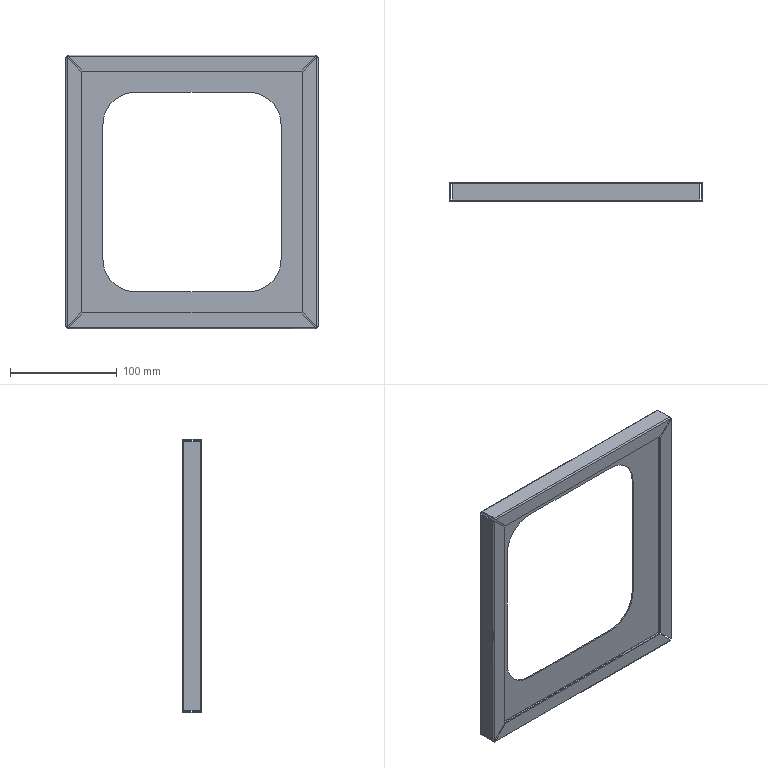Component | SolidWorks | Cover1-3XG1-2 | 1 solid | 78 faces | volume 70580 mm3 | plane 42 | cylinder 20 | spline 16 | commonest cylinder face diameters 2.5 x8 0.1 x8 60 x4